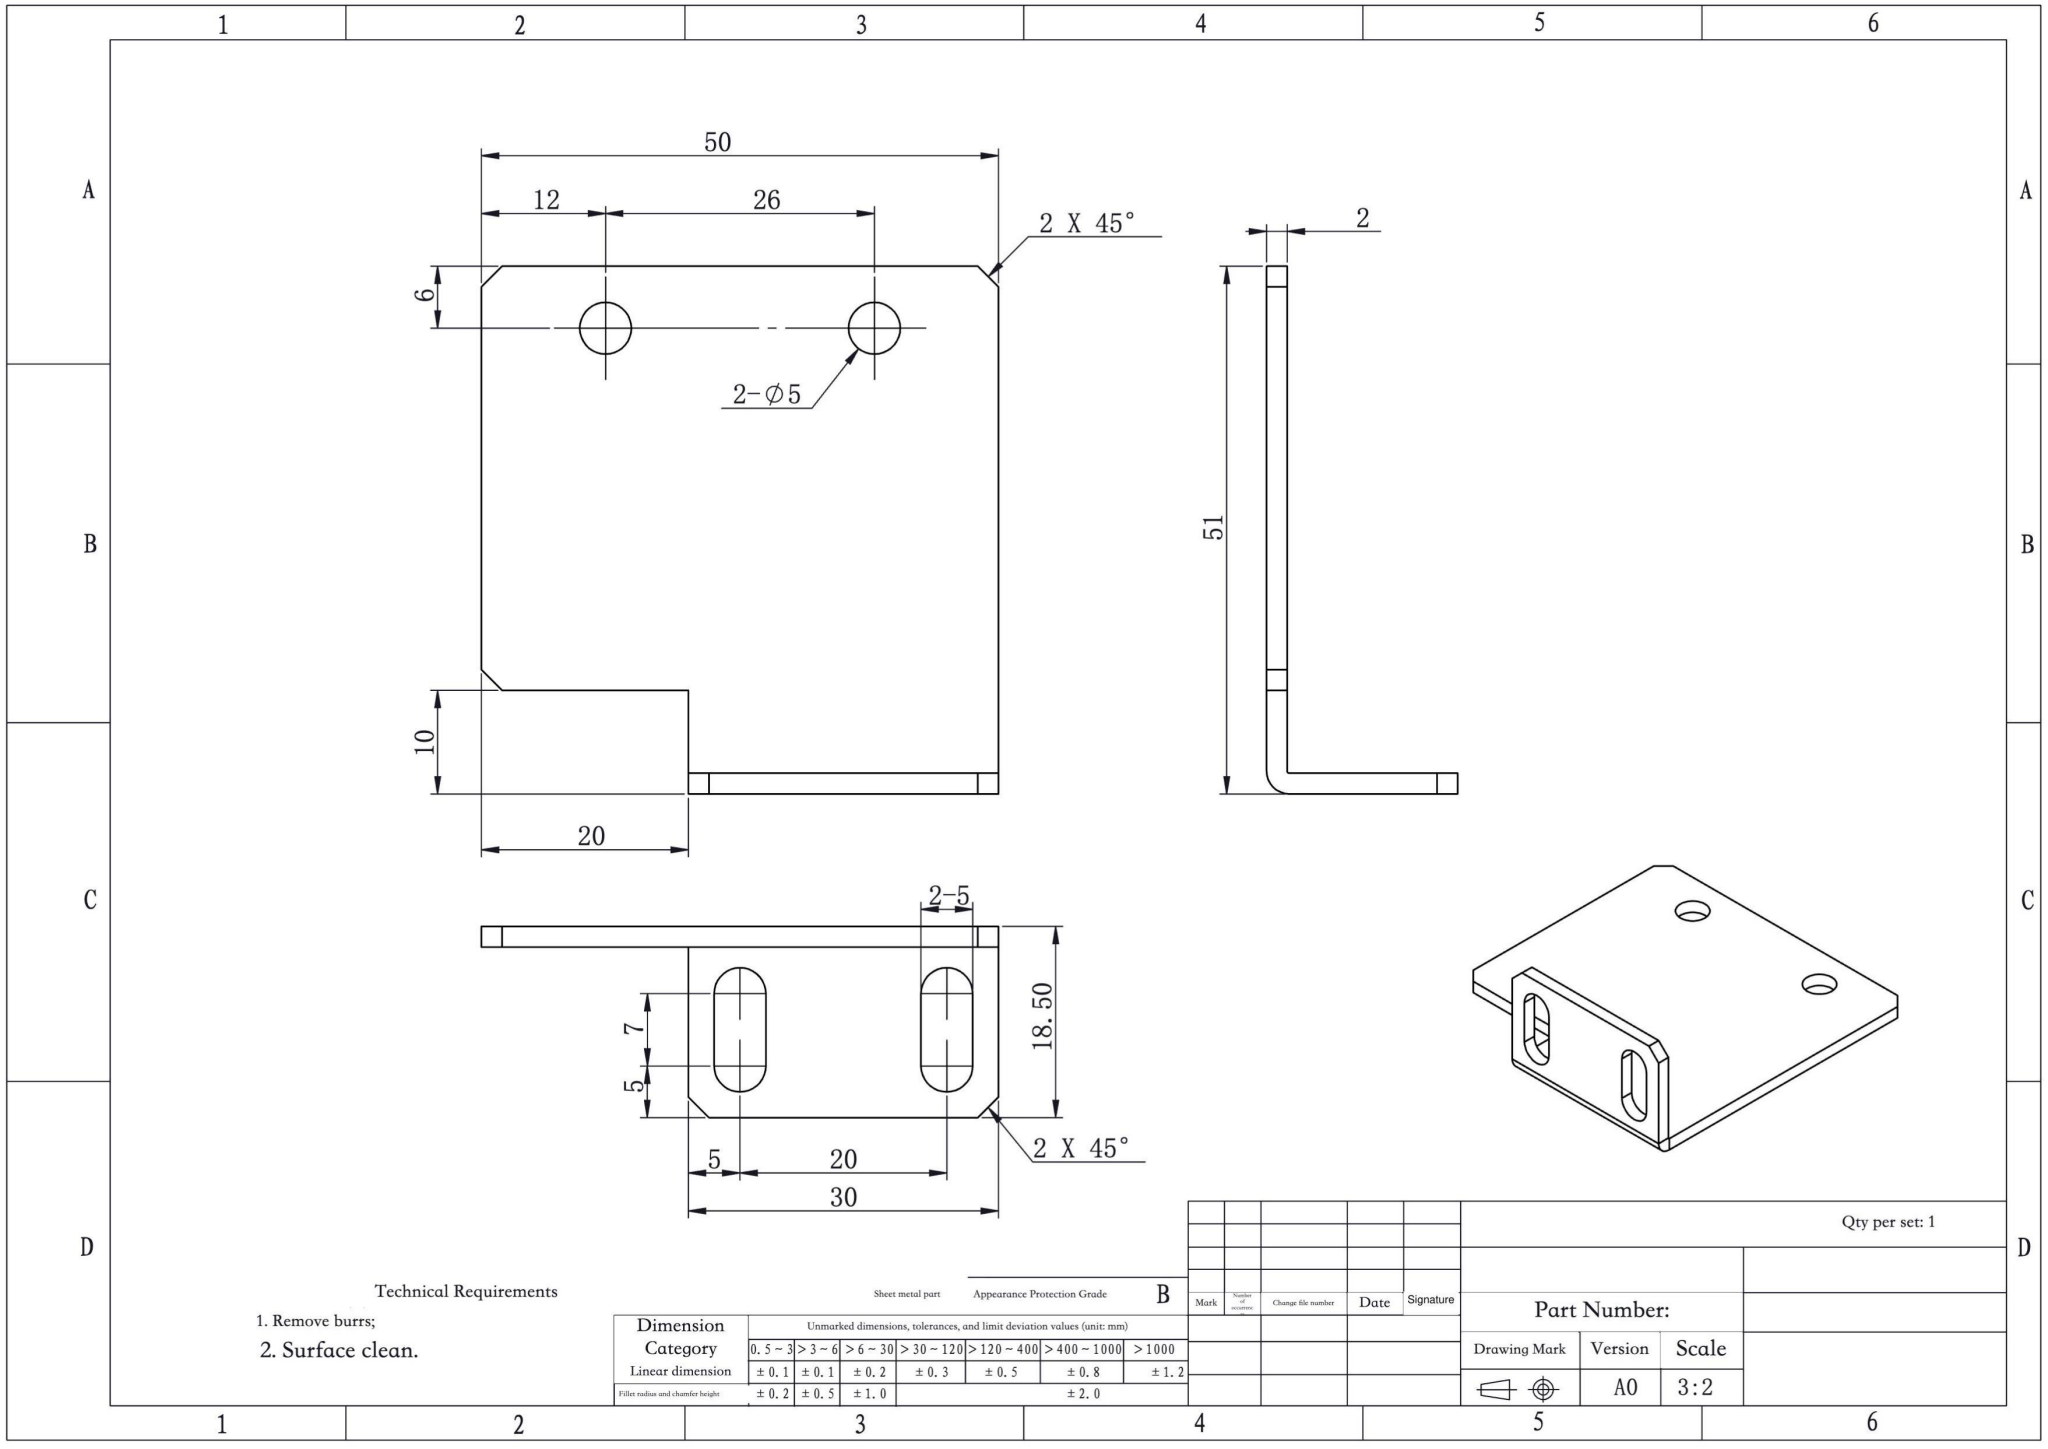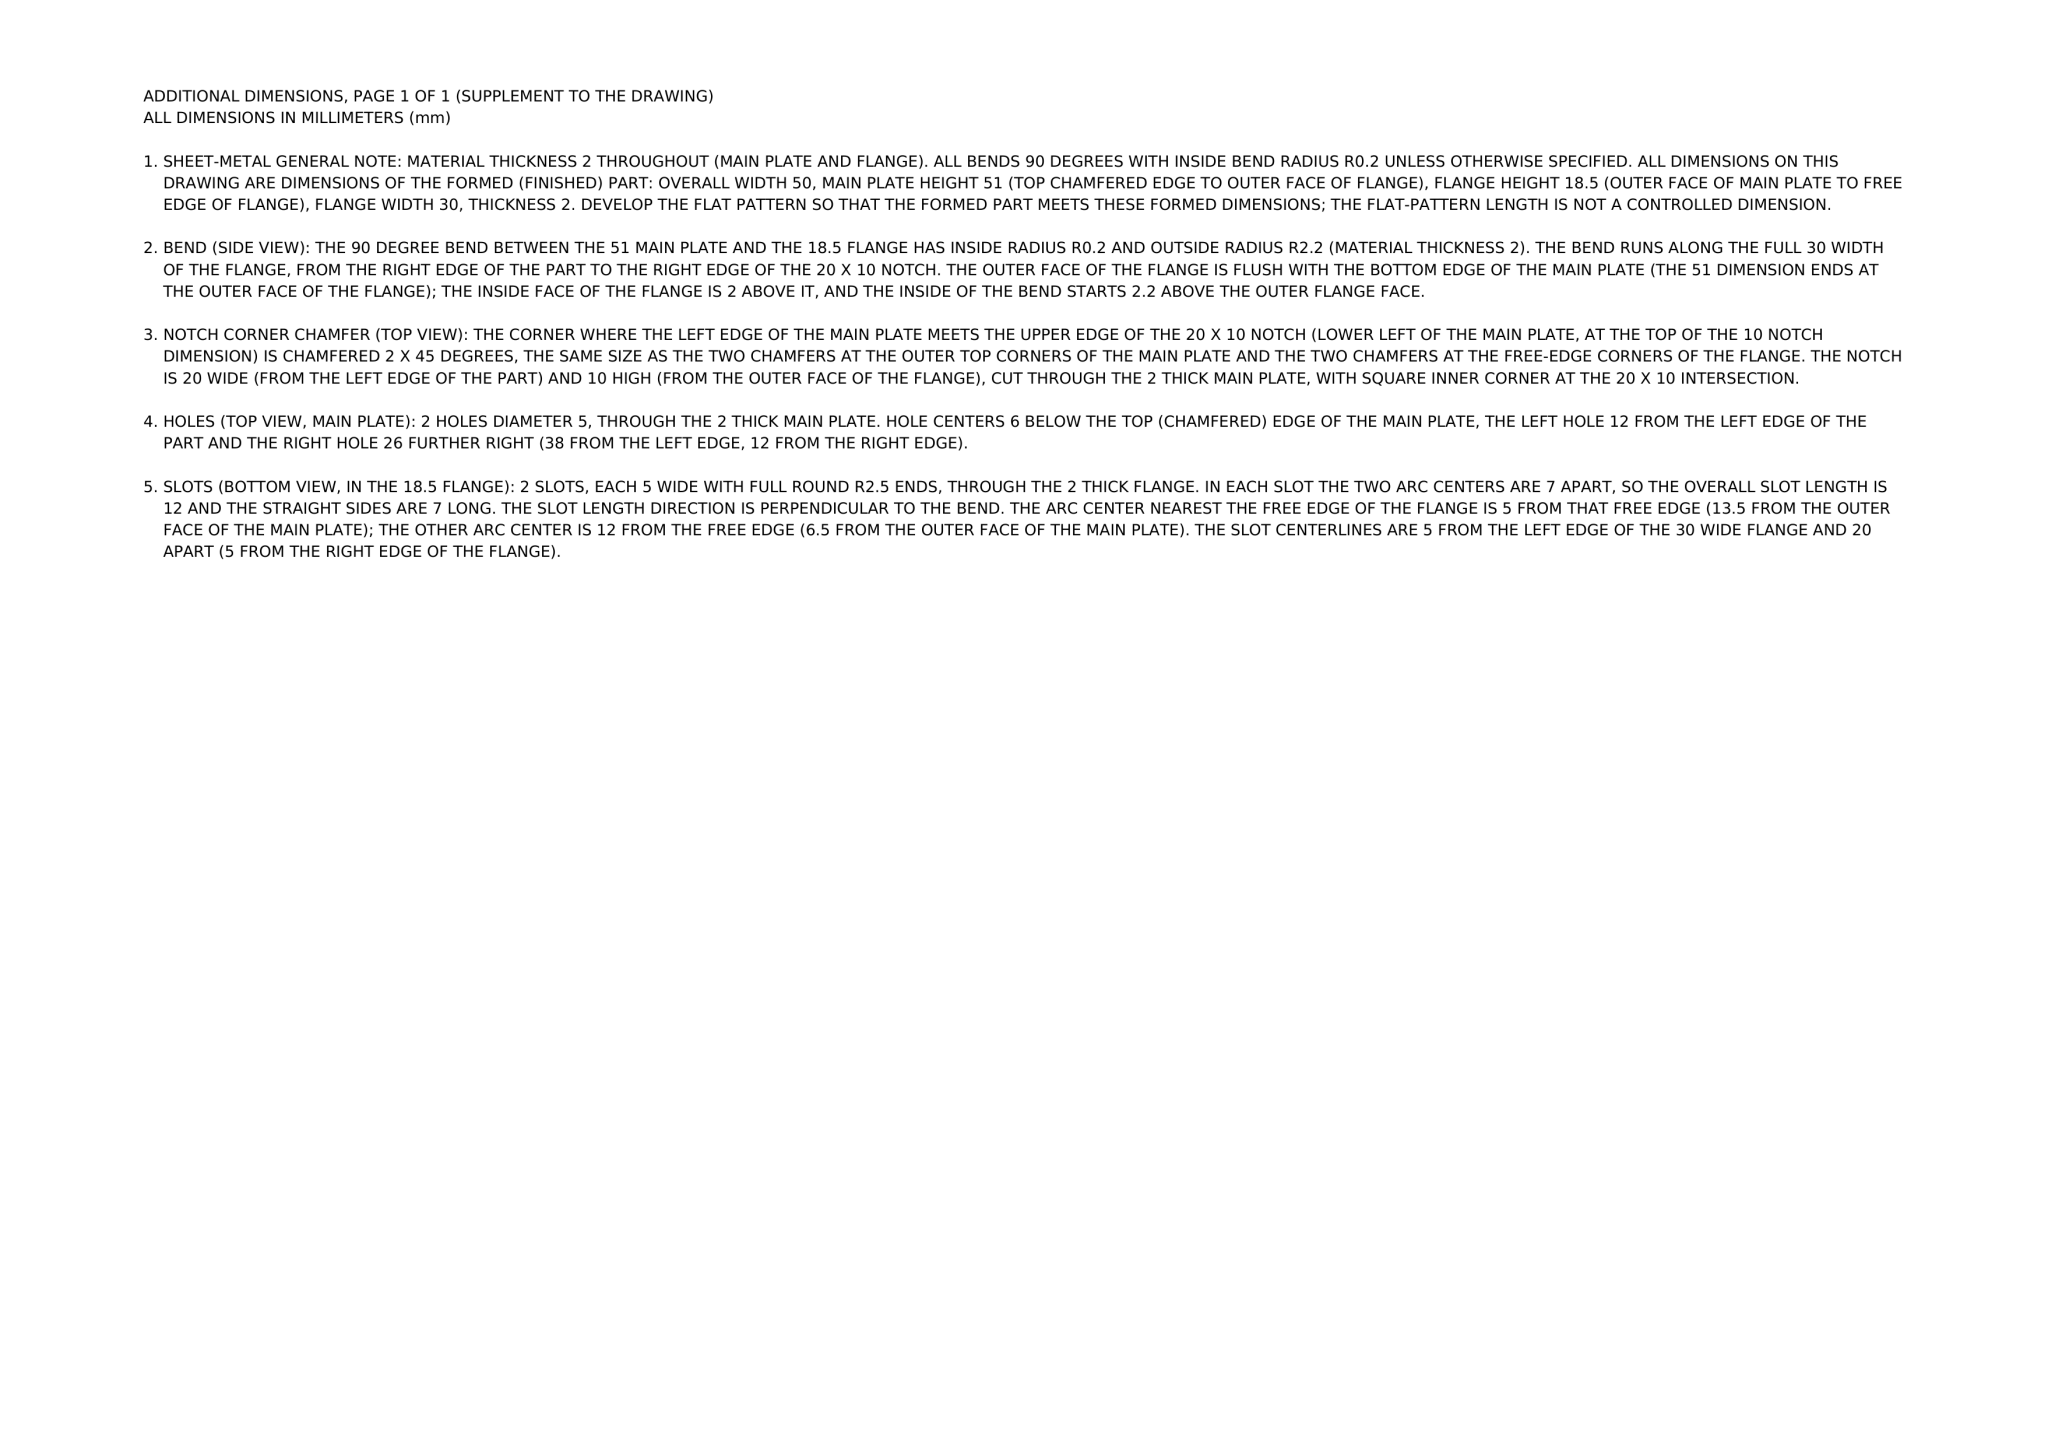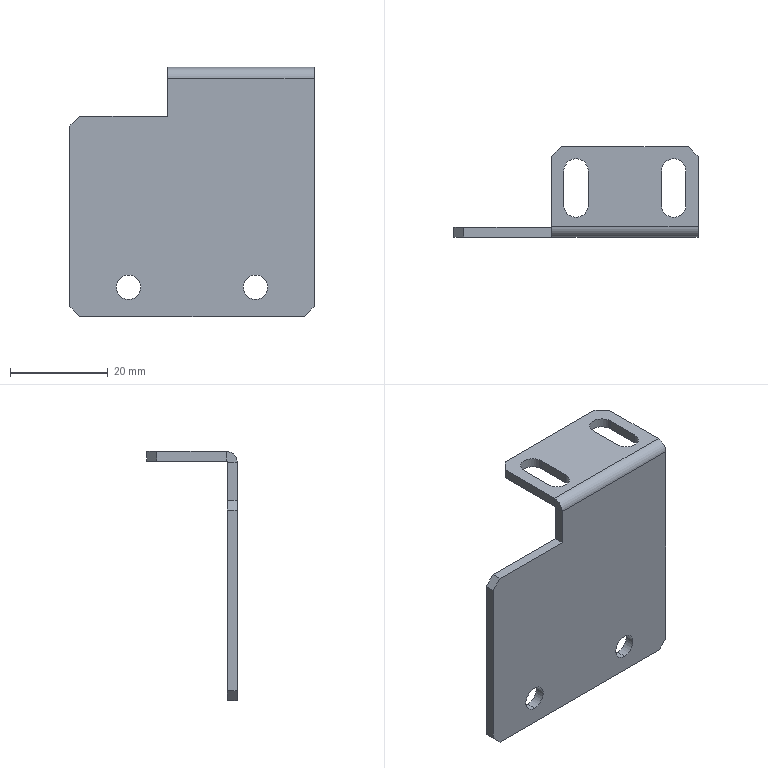Part | NX | mm | 1 solid | 33 faces | box 50 x 18.5 x 51 mm | volume 5342 mm3 | plane 23 | cylinder 10 | commonest cylinder face diameters 5 x8 4.4 x1 0.4 x1